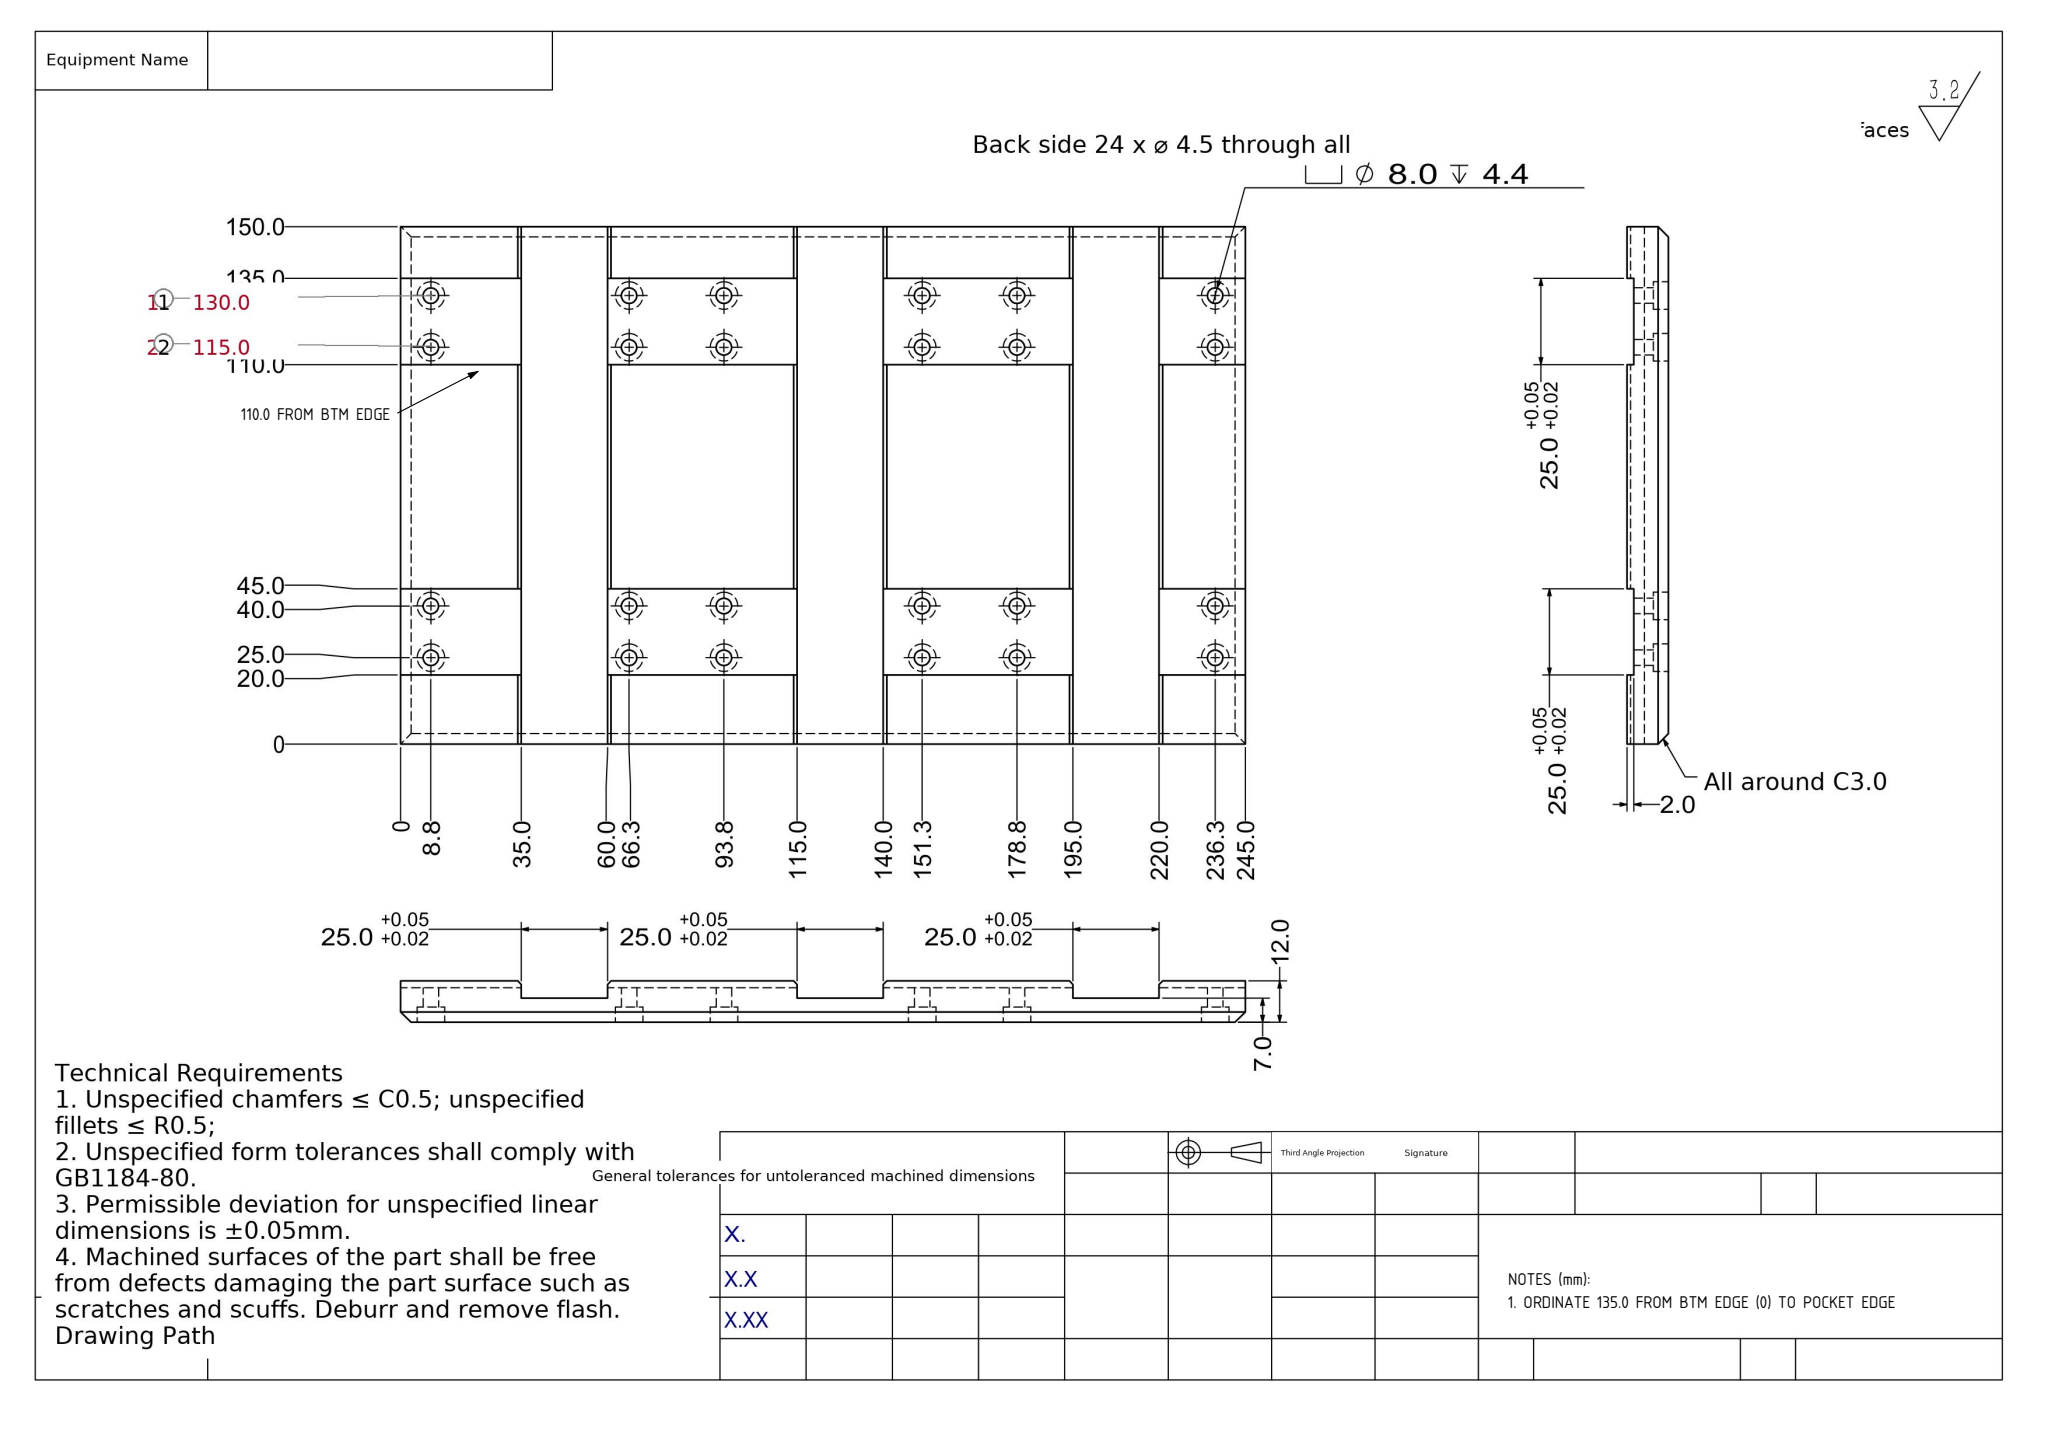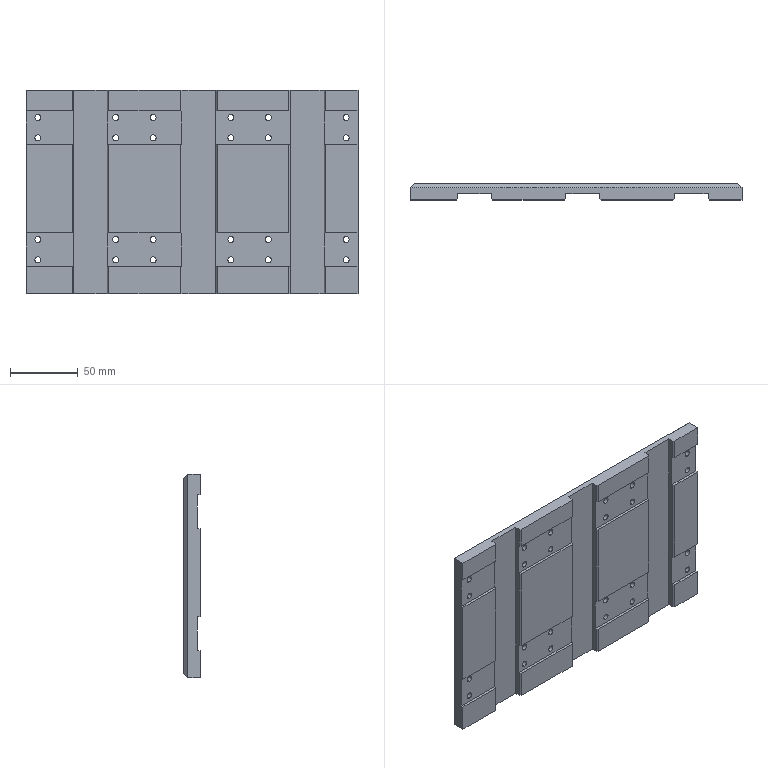Part | SolidWorks | mm | 1 solid | 192 faces | box 245 x 12 x 150 mm | volume 356485 mm3 | cylinder 96 | plane 96 | commonest cylinder face diameters 8 x48 4.5 x48
Drawing notes:
ORDINATE 135.0 FROM BTM EDGE (0) TO POCKET EDGE | from the solid: axis_planes z=135.0 (4 faces); datum z=0 bbox min
ORDINATE 110.0 FROM BTM EDGE (0) TO POCKET EDGE | from the solid: axis_planes z=110.0 (4 faces); datum z=0 bbox min
build123d program:
from build123d import *

# Parameters (mm, degrees)
SKETCH1_W                                       = 245
SKETCH1_H                                       = 150
BOSS_EXTRUDE1_DEPTH                             = 12
M4_HEX_SOCKET_HEAD_CAP_SCREW_CBORE1_D           = 4.5
M4_HEX_SOCKET_HEAD_CAP_SCREW_CBORE1_CBORE_D     = 8
M4_HEX_SOCKET_HEAD_CAP_SCREW_CBORE1_CBORE_DEPTH = 4.4
LPATTERN1_COUNT                                 = 3
LPATTERN1_PITCH                                 = 85
SKETCH5_W                                       = 245
SKETCH5_H                                       = 25
CUT_EXTRUDE1_DEPTH                              = 2
LPATTERN2_COUNT                                 = 2
LPATTERN2_PITCH                                 = 90
SKETCH6_W                                       = 25
SKETCH6_H                                       = 155
CUT_EXTRUDE2_DEPTH                              = 5
LPATTERN3_COUNT                                 = 3
LPATTERN3_PITCH                                 = 80
CHAMFER2_SIZE                                   = 3
CHAMFER3_SIZE                                   = 1


with BuildPart() as part:
    # Sketch1 → Boss-Extrude1 (new body)
    with BuildSketch(Plane(origin=(0, 0, 0), x_dir=(1, 0, 0), z_dir=(0, 1, 0))):
        Rectangle(SKETCH1_W, SKETCH1_H)
    extrude(amount=BOSS_EXTRUDE1_DEPTH)

    # M4 Hex Socket Head Cap Screw CBORE1 (through all)
    with Locations(Plane(origin=(0, 12, 0), x_dir=(1, 0, 0), z_dir=(0, 1, 0))):
        with Locations((-113.75, -55), (-113.75, -40), (-56.25, -55), (-56.25, -40), (-113.75, 35), (-113.75, 50), (-56.25, 35), (-56.25, 50)):
            m4_hex_socket_head_cap_screw_cbore1 = CounterBoreHole(M4_HEX_SOCKET_HEAD_CAP_SCREW_CBORE1_D / 2, M4_HEX_SOCKET_HEAD_CAP_SCREW_CBORE1_CBORE_D / 2, M4_HEX_SOCKET_HEAD_CAP_SCREW_CBORE1_CBORE_DEPTH)

    # LPattern1: M4 Hex Socket Head Cap Screw CBORE1 ×3
    with Locations(*[(i * LPATTERN1_PITCH, 0, 0) for i in range(1, LPATTERN1_COUNT)]):
        add(m4_hex_socket_head_cap_screw_cbore1, mode=Mode.SUBTRACT)

    # Sketch5 → Cut-Extrude1 (cut)
    with BuildSketch(Plane.XZ):
        with Locations((0, 47.5)):
            Rectangle(SKETCH5_W, SKETCH5_H)
    cut_extrude1 = extrude(amount=-CUT_EXTRUDE1_DEPTH, mode=Mode.SUBTRACT)

    # LPattern2: Cut-Extrude1 ×2
    with Locations(*[(0, 0, -i * LPATTERN2_PITCH) for i in range(1, LPATTERN2_COUNT)]):
        add(cut_extrude1, mode=Mode.SUBTRACT)

    # Sketch6 → Cut-Extrude2 (cut)
    with BuildSketch(Plane(origin=(0, 0, 0), x_dir=(-1, 0, 0), z_dir=(0, -1, 0))):
        with Locations((-85, -2.5)):
            Rectangle(SKETCH6_W, SKETCH6_H)
    cut_extrude2 = extrude(amount=-CUT_EXTRUDE2_DEPTH, mode=Mode.SUBTRACT)

    # LPattern3: Cut-Extrude2 ×3
    with Locations(*[(-i * LPATTERN3_PITCH, 0, 0) for i in range(1, LPATTERN3_COUNT)]):
        add(cut_extrude2, mode=Mode.SUBTRACT)

    # Chamfer2
    chamfer2_edges = [part.edges().sort_by_distance(p)[0] for p in [
        (-122.5, 12, 0),
        (0, 12, 75),
        (122.5, 12, 0),
        (0, 12, -75),
    ]]
    chamfer(chamfer2_edges, length=CHAMFER2_SIZE)

    # Chamfer3
    chamfer3_edges = [part.edges().sort_by_distance(p)[0] for p in [
        (97.5, 0, 67.5),
        (72.5, 0, 67.5),
        (97.5, 0, 2.5),
        (72.5, 0, 2.5),
        (97.5, 0, -65),
        (72.5, 0, -65),
        (17.5, 0, 67.5),
        (-7.5, 0, 67.5),
        (17.5, 0, 2.5),
        (-7.5, 0, 2.5),
        (17.5, 0, -65),
        (-7.5, 0, -65),
        (-62.5, 0, 67.5),
        (-87.5, 0, 67.5),
        (-62.5, 0, 2.5),
        (-87.5, 0, 2.5),
        (-62.5, 0, -65),
        (-87.5, 0, -65),
    ]]
    chamfer(chamfer3_edges, length=CHAMFER3_SIZE)


solid = part.part